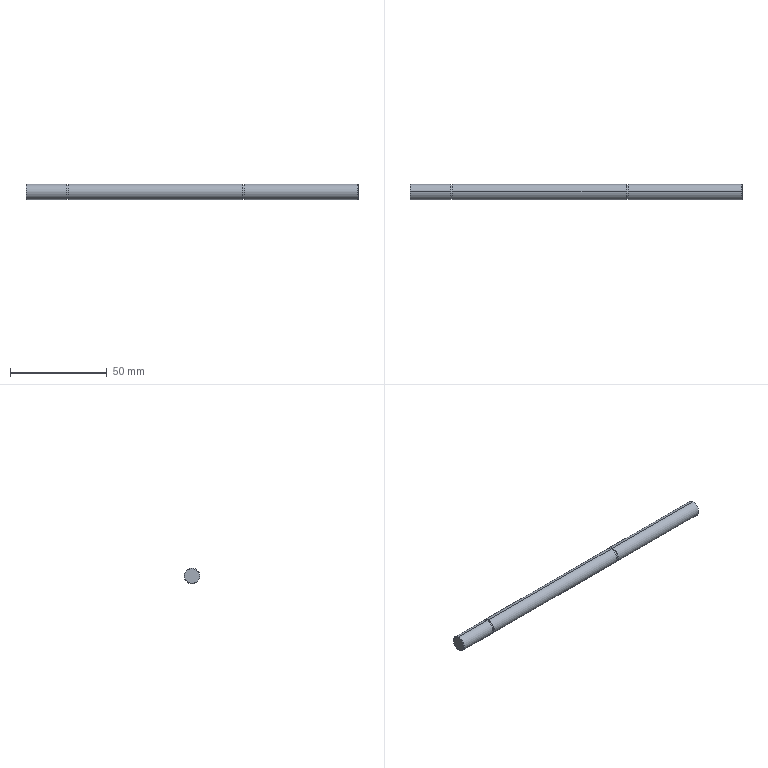Component | SolidWorks | 04-003DriveShaft-1 | 1 solid | 20 faces | box 172 x 8 x 8 mm | volume 8630 mm3 | cylinder 10 | plane 6 | cone 4 | commonest cylinder face diameters 8 x6 7.4 x4
build123d program:
from build123d import *

# Parameters (mm, degrees)
SKETCH1_R           = 4
BOSS_EXTRUDE1_DEPTH = 172
CHAMFER1_SIZE       = 0.2
SKETCH2_W           = 1
SKETCH2_H           = 0.3


with BuildPart() as part:
    # Sketch1 → Boss-Extrude1 (new body)
    with BuildSketch(Plane(origin=(0, 0, 0), x_dir=(0, 0, -1), z_dir=(1, 0, 0))):
        Circle(SKETCH1_R)
    extrude(amount=BOSS_EXTRUDE1_DEPTH)

    # Chamfer1
    chamfer1_edges = [part.edges().sort_by_distance(p)[0] for p in [
        (0, 0, 4),
        (172, 0, 4),
    ]]
    chamfer(chamfer1_edges, length=CHAMFER1_SIZE)

    # Sketch2 → Cut-Revolve1 (revolve, cut)
    with BuildSketch(Plane(origin=(0, 0, 0), x_dir=(1, 0, 0), z_dir=(0, 1, 0)), mode=Mode.PRIVATE) as cut_revolve1_sk:
        with Locations((21.5, 3.85)):
            Rectangle(SKETCH2_W, SKETCH2_H)
        with Locations((112.5, 3.85)):
            Rectangle(SKETCH2_W, SKETCH2_H)
    revolve(cut_revolve1_sk.sketch.rotate(Axis((0, 0, 0), (1, 0, 0)), 180), axis=Axis((0, 0, 0), (1, 0, 0)), mode=Mode.SUBTRACT)


solid = part.part

# Placed as in the assembly
solid = solid.moved(Location((-2.274, -5.336, 80.465), (0, 0, 0)))
STEP:
#1=COLOUR_RGB('',0.7922,0.8196,0.9333);
#2=FILL_AREA_STYLE_COLOUR('',#1);
#3=FILL_AREA_STYLE('',(#2));
#4=SURFACE_STYLE_FILL_AREA(#3);
#5=SURFACE_SIDE_STYLE('',(#4));
#6=SURFACE_STYLE_USAGE(.BOTH.,#5);
#7=PRESENTATION_STYLE_ASSIGNMENT((#6));
#8=CARTESIAN_POINT('',(6.674,-0.2215,3.011));
#9=VERTEX_POINT('',#8);
#10=CARTESIAN_POINT('',(6.674,-0.1986,3.325));
#11=VERTEX_POINT('',#10);
#12=CARTESIAN_POINT('',(6.674,-0.2101,3.168));
#13=DIRECTION('',(-1.,0.,0.));
#14=DIRECTION('',(0.,0.07282,0.9973));
#15=AXIS2_PLACEMENT_3D('',#12,#13,#14);
#16=CIRCLE('',#15,0.1575);
#17=EDGE_CURVE('',#9,#11,#16,.T.);
#18=ORIENTED_EDGE('',*,*,#17,.T.);
#19=CARTESIAN_POINT('',(4.359,-0.1986,3.325));
#20=VERTEX_POINT('',#19);
#21=CARTESIAN_POINT('',(6.682,-0.1986,3.325));
#22=DIRECTION('',(-1.,0.,0.));
#23=VECTOR('',#22,39.37);
#24=LINE('',#21,#23);
#25=EDGE_CURVE('',#11,#20,#24,.T.);
#26=ORIENTED_EDGE('',*,*,#25,.T.);
#27=CARTESIAN_POINT('',(4.359,-0.2215,3.011));
#28=VERTEX_POINT('',#27);
#29=CARTESIAN_POINT('',(4.359,-0.2101,3.168));
#30=DIRECTION('',(-1.,0.,0.));
#31=DIRECTION('',(0.,-0.07282,-0.9973));
#32=AXIS2_PLACEMENT_3D('',#29,#30,#31);
#33=CIRCLE('',#32,0.1575);
#34=EDGE_CURVE('',#28,#20,#33,.T.);
#35=ORIENTED_EDGE('',*,*,#34,.F.);
#36=CARTESIAN_POINT('',(6.682,-0.2215,3.011));
#37=DIRECTION('',(-1.,0.,0.));
#38=VECTOR('',#37,39.37);
#39=LINE('',#36,#38);
#40=EDGE_CURVE('',#9,#28,#39,.T.);
#41=ORIENTED_EDGE('',*,*,#40,.F.);
#42=EDGE_LOOP('',(#18,#26,#35,#41));
#43=FACE_OUTER_BOUND('',#42,.T.);
#44=CARTESIAN_POINT('',(6.682,-0.2101,3.168));
#45=DIRECTION('',(-1.,0.,0.));
#46=DIRECTION('',(0.,-0.07282,-0.9973));
#47=AXIS2_PLACEMENT_3D('',#44,#45,#46);
#48=CYLINDRICAL_SURFACE('',#47,0.1575);
#49=ADVANCED_FACE('',(#43),#48,.T.);
#50=CARTESIAN_POINT('',(6.682,-0.1992,3.317));
#51=VERTEX_POINT('',#50);
#52=CARTESIAN_POINT('',(6.682,-0.221,3.019));
#53=VERTEX_POINT('',#52);
#54=CARTESIAN_POINT('',(6.682,-0.2101,3.168));
#55=DIRECTION('',(1.,0.,0.));
#56=DIRECTION('',(0.,0.07282,0.9973));
#57=AXIS2_PLACEMENT_3D('',#54,#55,#56);
#58=CIRCLE('',#57,0.1496);
#59=EDGE_CURVE('',#51,#53,#58,.T.);
#60=ORIENTED_EDGE('',*,*,#59,.F.);
#61=CARTESIAN_POINT('',(6.682,-0.1992,3.317));
#62=DIRECTION('',(-0.7071,0.05149,0.7052));
#63=VECTOR('',#62,39.37);
#64=LINE('',#61,#63);
#65=EDGE_CURVE('',#51,#11,#64,.T.);
#66=ORIENTED_EDGE('',*,*,#65,.T.);
#67=ORIENTED_EDGE('',*,*,#17,.F.);
#68=CARTESIAN_POINT('',(6.682,-0.221,3.019));
#69=DIRECTION('',(-0.7071,-0.05149,-0.7052));
#70=VECTOR('',#69,39.37);
#71=LINE('',#68,#70);
#72=EDGE_CURVE('',#53,#9,#71,.T.);
#73=ORIENTED_EDGE('',*,*,#72,.F.);
#74=EDGE_LOOP('',(#60,#66,#67,#73));
#75=FACE_OUTER_BOUND('',#74,.T.);
#76=CARTESIAN_POINT('',(6.682,-0.2101,3.168));
#77=DIRECTION('',(-1.,0.,0.));
#78=DIRECTION('',(0.,-0.07282,-0.9973));
#79=AXIS2_PLACEMENT_3D('',#76,#77,#78);
#80=CONICAL_SURFACE('',#79,0.1496,0.7854);
#81=ADVANCED_FACE('',(#75),#80,.T.);
#82=CARTESIAN_POINT('',(4.359,-0.2207,3.023));
#83=VERTEX_POINT('',#82);
#84=CARTESIAN_POINT('',(4.359,-0.1995,3.313));
#85=VERTEX_POINT('',#84);
#86=CARTESIAN_POINT('',(4.359,-0.2101,3.168));
#87=DIRECTION('',(-1.,0.,0.));
#88=DIRECTION('',(0.,-0.07282,-0.9973));
#89=AXIS2_PLACEMENT_3D('',#86,#87,#88);
#90=CIRCLE('',#89,0.1457);
#91=EDGE_CURVE('',#83,#85,#90,.T.);
#92=ORIENTED_EDGE('',*,*,#91,.T.);
#93=CARTESIAN_POINT('',(4.32,-0.1995,3.313));
#94=VERTEX_POINT('',#93);
#95=CARTESIAN_POINT('',(-0.08951,-0.1995,3.313));
#96=DIRECTION('',(-1.,0.,0.));
#97=VECTOR('',#96,39.37);
#98=LINE('',#95,#97);
#99=EDGE_CURVE('',#85,#94,#98,.T.);
#100=ORIENTED_EDGE('',*,*,#99,.T.);
#101=CARTESIAN_POINT('',(4.32,-0.2207,3.023));
#102=VERTEX_POINT('',#101);
#103=CARTESIAN_POINT('',(4.32,-0.2101,3.168));
#104=DIRECTION('',(-1.,0.,0.));
#105=DIRECTION('',(0.,-0.07282,-0.9973));
#106=AXIS2_PLACEMENT_3D('',#103,#104,#105);
#107=CIRCLE('',#106,0.1457);
#108=EDGE_CURVE('',#102,#94,#107,.T.);
#109=ORIENTED_EDGE('',*,*,#108,.F.);
#110=CARTESIAN_POINT('',(-0.08951,-0.2207,3.023));
#111=DIRECTION('',(-1.,0.,0.));
#112=VECTOR('',#111,39.37);
#113=LINE('',#110,#112);
#114=EDGE_CURVE('',#83,#102,#113,.T.);
#115=ORIENTED_EDGE('',*,*,#114,.F.);
#116=EDGE_LOOP('',(#92,#100,#109,#115));
#117=FACE_OUTER_BOUND('',#116,.T.);
#118=CARTESIAN_POINT('',(-0.08951,-0.2101,3.168));
#119=DIRECTION('',(-1.,0.,0.));
#120=DIRECTION('',(0.,-0.07282,-0.9973));
#121=AXIS2_PLACEMENT_3D('',#118,#119,#120);
#122=CYLINDRICAL_SURFACE('',#121,0.1457);
#123=ADVANCED_FACE('',(#117),#122,.T.);
#124=CARTESIAN_POINT('',(4.32,-0.2215,3.011));
#125=VERTEX_POINT('',#124);
#126=CARTESIAN_POINT('',(4.32,-0.1986,3.325));
#127=VERTEX_POINT('',#126);
#128=CARTESIAN_POINT('',(4.32,-0.2101,3.168));
#129=DIRECTION('',(-1.,0.,0.));
#130=DIRECTION('',(0.,-0.07282,-0.9973));
#131=AXIS2_PLACEMENT_3D('',#128,#129,#130);
#132=CIRCLE('',#131,0.1575);
#133=EDGE_CURVE('',#125,#127,#132,.T.);
#134=ORIENTED_EDGE('',*,*,#133,.T.);
#135=CARTESIAN_POINT('',(0.7766,-0.1986,3.325));
#136=VERTEX_POINT('',#135);
#137=CARTESIAN_POINT('',(6.682,-0.1986,3.325));
#138=DIRECTION('',(-1.,0.,0.));
#139=VECTOR('',#138,39.37);
#140=LINE('',#137,#139);
#141=EDGE_CURVE('',#127,#136,#140,.T.);
#142=ORIENTED_EDGE('',*,*,#141,.T.);
#143=CARTESIAN_POINT('',(0.7766,-0.2215,3.011));
#144=VERTEX_POINT('',#143);
#145=CARTESIAN_POINT('',(0.7766,-0.2101,3.168));
#146=DIRECTION('',(-1.,0.,0.));
#147=DIRECTION('',(0.,-0.07282,-0.9973));
#148=AXIS2_PLACEMENT_3D('',#145,#146,#147);
#149=CIRCLE('',#148,0.1575);
#150=EDGE_CURVE('',#144,#136,#149,.T.);
#151=ORIENTED_EDGE('',*,*,#150,.F.);
#152=CARTESIAN_POINT('',(6.682,-0.2215,3.011));
#153=DIRECTION('',(-1.,0.,0.));
#154=VECTOR('',#153,39.37);
#155=LINE('',#152,#154);
#156=EDGE_CURVE('',#125,#144,#155,.T.);
#157=ORIENTED_EDGE('',*,*,#156,.F.);
#158=EDGE_LOOP('',(#134,#142,#151,#157));
#159=FACE_OUTER_BOUND('',#158,.T.);
#160=CARTESIAN_POINT('',(6.682,-0.2101,3.168));
#161=DIRECTION('',(-1.,0.,0.));
#162=DIRECTION('',(0.,-0.07282,-0.9973));
#163=AXIS2_PLACEMENT_3D('',#160,#161,#162);
#164=CYLINDRICAL_SURFACE('',#163,0.1575);
#165=ADVANCED_FACE('',(#159),#164,.T.);
#166=CARTESIAN_POINT('',(0.7766,-0.2207,3.023));
#167=VERTEX_POINT('',#166);
#168=CARTESIAN_POINT('',(0.7766,-0.1995,3.313));
#169=VERTEX_POINT('',#168);
#170=CARTESIAN_POINT('',(0.7766,-0.2101,3.168));
#171=DIRECTION('',(-1.,0.,0.));
#172=DIRECTION('',(0.,-0.07282,-0.9973));
#173=AXIS2_PLACEMENT_3D('',#170,#171,#172);
#174=CIRCLE('',#173,0.1457);
#175=EDGE_CURVE('',#167,#169,#174,.T.);
#176=ORIENTED_EDGE('',*,*,#175,.T.);
#177=CARTESIAN_POINT('',(0.7373,-0.1995,3.313));
#178=VERTEX_POINT('',#177);
#179=CARTESIAN_POINT('',(-0.08951,-0.1995,3.313));
#180=DIRECTION('',(-1.,0.,0.));
#181=VECTOR('',#180,39.37);
#182=LINE('',#179,#181);
#183=EDGE_CURVE('',#169,#178,#182,.T.);
#184=ORIENTED_EDGE('',*,*,#183,.T.);
#185=CARTESIAN_POINT('',(0.7373,-0.2207,3.023));
#186=VERTEX_POINT('',#185);
#187=CARTESIAN_POINT('',(0.7373,-0.2101,3.168));
#188=DIRECTION('',(-1.,0.,0.));
#189=DIRECTION('',(0.,-0.07282,-0.9973));
#190=AXIS2_PLACEMENT_3D('',#187,#188,#189);
#191=CIRCLE('',#190,0.1457);
#192=EDGE_CURVE('',#186,#178,#191,.T.);
#193=ORIENTED_EDGE('',*,*,#192,.F.);
#194=CARTESIAN_POINT('',(-0.08951,-0.2207,3.023));
#195=DIRECTION('',(-1.,0.,0.));
#196=VECTOR('',#195,39.37);
#197=LINE('',#194,#196);
#198=EDGE_CURVE('',#167,#186,#197,.T.);
#199=ORIENTED_EDGE('',*,*,#198,.F.);
#200=EDGE_LOOP('',(#176,#184,#193,#199));
#201=FACE_OUTER_BOUND('',#200,.T.);
#202=CARTESIAN_POINT('',(-0.08951,-0.2101,3.168));
#203=DIRECTION('',(-1.,0.,0.));
#204=DIRECTION('',(0.,-0.07282,-0.9973));
#205=AXIS2_PLACEMENT_3D('',#202,#203,#204);
#206=CYLINDRICAL_SURFACE('',#205,0.1457);
#207=ADVANCED_FACE('',(#201),#206,.T.);
#208=CARTESIAN_POINT('',(-0.08951,-0.221,3.019));
#209=VERTEX_POINT('',#208);
#210=CARTESIAN_POINT('',(-0.08951,-0.1992,3.317));
#211=VERTEX_POINT('',#210);
#212=CARTESIAN_POINT('',(-0.08951,-0.2101,3.168));
#213=DIRECTION('',(-1.,0.,0.));
#214=DIRECTION('',(0.,0.07282,0.9973));
#215=AXIS2_PLACEMENT_3D('',#212,#213,#214);
#216=CIRCLE('',#215,0.1496);
#217=EDGE_CURVE('',#209,#211,#216,.T.);
#218=ORIENTED_EDGE('',*,*,#217,.F.);
#219=CARTESIAN_POINT('',(-0.08164,-0.2215,3.011));
#220=VERTEX_POINT('',#219);
#221=CARTESIAN_POINT('',(-0.08164,-0.2215,3.011));
#222=DIRECTION('',(0.7071,-0.05149,-0.7052));
#223=VECTOR('',#222,39.37);
#224=LINE('',#221,#223);
#225=EDGE_CURVE('',#209,#220,#224,.T.);
#226=ORIENTED_EDGE('',*,*,#225,.T.);
#227=CARTESIAN_POINT('',(-0.08164,-0.1986,3.325));
#228=VERTEX_POINT('',#227);
#229=CARTESIAN_POINT('',(-0.08164,-0.2101,3.168));
#230=DIRECTION('',(1.,0.,0.));
#231=DIRECTION('',(0.,0.07282,0.9973));
#232=AXIS2_PLACEMENT_3D('',#229,#230,#231);
#233=CIRCLE('',#232,0.1575);
#234=EDGE_CURVE('',#228,#220,#233,.T.);
#235=ORIENTED_EDGE('',*,*,#234,.F.);
#236=CARTESIAN_POINT('',(-0.08164,-0.1986,3.325));
#237=DIRECTION('',(0.7071,0.05149,0.7052));
#238=VECTOR('',#237,39.37);
#239=LINE('',#236,#238);
#240=EDGE_CURVE('',#211,#228,#239,.T.);
#241=ORIENTED_EDGE('',*,*,#240,.F.);
#242=EDGE_LOOP('',(#218,#226,#235,#241));
#243=FACE_OUTER_BOUND('',#242,.T.);
#244=CARTESIAN_POINT('',(-0.08164,-0.2101,3.168));
#245=DIRECTION('',(1.,0.,0.));
#246=DIRECTION('',(0.,0.07282,0.9973));
#247=AXIS2_PLACEMENT_3D('',#244,#245,#246);
#248=CONICAL_SURFACE('',#247,0.1575,0.7854);
#249=ADVANCED_FACE('',(#243),#248,.T.);
#250=CARTESIAN_POINT('',(0.7373,-0.2215,3.011));
#251=VERTEX_POINT('',#250);
#252=CARTESIAN_POINT('',(0.7373,-0.1986,3.325));
#253=VERTEX_POINT('',#252);
#254=CARTESIAN_POINT('',(0.7373,-0.2101,3.168));
#255=DIRECTION('',(-1.,0.,0.));
#256=DIRECTION('',(0.,-0.07282,-0.9973));
#257=AXIS2_PLACEMENT_3D('',#254,#255,#256);
#258=CIRCLE('',#257,0.1575);
#259=EDGE_CURVE('',#251,#253,#258,.T.);
#260=ORIENTED_EDGE('',*,*,#259,.T.);
#261=CARTESIAN_POINT('',(6.682,-0.1986,3.325));
#262=DIRECTION('',(-1.,0.,0.));
#263=VECTOR('',#262,39.37);
#264=LINE('',#261,#263);
#265=EDGE_CURVE('',#253,#228,#264,.T.);
#266=ORIENTED_EDGE('',*,*,#265,.T.);
#267=ORIENTED_EDGE('',*,*,#234,.T.);
#268=CARTESIAN_POINT('',(6.682,-0.2215,3.011));
#269=DIRECTION('',(-1.,0.,0.));
#270=VECTOR('',#269,39.37);
#271=LINE('',#268,#270);
#272=EDGE_CURVE('',#251,#220,#271,.T.);
#273=ORIENTED_EDGE('',*,*,#272,.F.);
#274=EDGE_LOOP('',(#260,#266,#267,#273));
#275=FACE_OUTER_BOUND('',#274,.T.);
#276=CARTESIAN_POINT('',(6.682,-0.2101,3.168));
#277=DIRECTION('',(-1.,0.,0.));
#278=DIRECTION('',(0.,-0.07282,-0.9973));
#279=AXIS2_PLACEMENT_3D('',#276,#277,#278);
#280=CYLINDRICAL_SURFACE('',#279,0.1575);
#281=ADVANCED_FACE('',(#275),#280,.T.);
#282=ORIENTED_EDGE('',*,*,#265,.F.);
#283=CARTESIAN_POINT('',(0.7373,-0.2101,3.168));
#284=DIRECTION('',(-1.,0.,0.));
#285=DIRECTION('',(0.,-0.07282,-0.9973));
#286=AXIS2_PLACEMENT_3D('',#283,#284,#285);
#287=CIRCLE('',#286,0.1575);
#288=EDGE_CURVE('',#253,#251,#287,.T.);
#289=ORIENTED_EDGE('',*,*,#288,.T.);
#290=ORIENTED_EDGE('',*,*,#272,.T.);
#291=CARTESIAN_POINT('',(-0.08164,-0.2101,3.168));
#292=DIRECTION('',(1.,0.,0.));
#293=DIRECTION('',(0.,0.07282,0.9973));
#294=AXIS2_PLACEMENT_3D('',#291,#292,#293);
#295=CIRCLE('',#294,0.1575);
#296=EDGE_CURVE('',#220,#228,#295,.T.);
#297=ORIENTED_EDGE('',*,*,#296,.T.);
#298=EDGE_LOOP('',(#282,#289,#290,#297));
#299=FACE_OUTER_BOUND('',#298,.T.);
#300=CARTESIAN_POINT('',(6.682,-0.2101,3.168));
#301=DIRECTION('',(-1.,0.,0.));
#302=DIRECTION('',(0.,-0.07282,-0.9973));
#303=AXIS2_PLACEMENT_3D('',#300,#301,#302);
#304=CYLINDRICAL_SURFACE('',#303,0.1575);
#305=ADVANCED_FACE('',(#299),#304,.T.);
#306=CARTESIAN_POINT('',(-0.08951,-0.2101,3.168));
#307=DIRECTION('',(-1.,0.,0.));
#308=DIRECTION('',(0.,0.07282,0.9973));
#309=AXIS2_PLACEMENT_3D('',#306,#307,#308);
#310=CIRCLE('',#309,0.1496);
#311=EDGE_CURVE('',#211,#209,#310,.T.);
#312=ORIENTED_EDGE('',*,*,#311,.T.);
#313=ORIENTED_EDGE('',*,*,#217,.T.);
#314=EDGE_LOOP('',(#312,#313));
#315=FACE_OUTER_BOUND('',#314,.T.);
#316=CARTESIAN_POINT('',(-0.08951,-0.2101,3.168));
#317=DIRECTION('',(1.,0.,0.));
#318=DIRECTION('',(0.,0.07282,0.9973));
#319=AXIS2_PLACEMENT_3D('',#316,#317,#318);
#320=PLANE('',#319);
#321=ADVANCED_FACE('',(#315),#320,.F.);
#322=ORIENTED_EDGE('',*,*,#225,.F.);
#323=ORIENTED_EDGE('',*,*,#311,.F.);
#324=ORIENTED_EDGE('',*,*,#240,.T.);
#325=ORIENTED_EDGE('',*,*,#296,.F.);
#326=EDGE_LOOP('',(#322,#323,#324,#325));
#327=FACE_OUTER_BOUND('',#326,.T.);
#328=CARTESIAN_POINT('',(-0.08164,-0.2101,3.168));
#329=DIRECTION('',(1.,0.,0.));
#330=DIRECTION('',(0.,0.07282,0.9973));
#331=AXIS2_PLACEMENT_3D('',#328,#329,#330);
#332=CONICAL_SURFACE('',#331,0.1575,0.7854);
#333=ADVANCED_FACE('',(#327),#332,.T.);
#334=ORIENTED_EDGE('',*,*,#192,.T.);
#335=CARTESIAN_POINT('',(0.7373,-0.2101,3.168));
#336=DIRECTION('',(-1.,0.,0.));
#337=DIRECTION('',(0.,-0.07282,-0.9973));
#338=AXIS2_PLACEMENT_3D('',#335,#336,#337);
#339=CIRCLE('',#338,0.1457);
#340=EDGE_CURVE('',#178,#186,#339,.T.);
#341=ORIENTED_EDGE('',*,*,#340,.T.);
#342=EDGE_LOOP('',(#334,#341));
#343=FACE_BOUND('',#342,.T.);
#344=ORIENTED_EDGE('',*,*,#259,.F.);
#345=ORIENTED_EDGE('',*,*,#288,.F.);
#346=EDGE_LOOP('',(#344,#345));
#347=FACE_OUTER_BOUND('',#346,.T.);
#348=CARTESIAN_POINT('',(0.7373,-0.1986,3.325));
#349=DIRECTION('',(1.,0.,0.));
#350=DIRECTION('',(0.,0.07282,0.9973));
#351=AXIS2_PLACEMENT_3D('',#348,#349,#350);
#352=PLANE('',#351);
#353=ADVANCED_FACE('',(#343,#347),#352,.T.);
#354=ORIENTED_EDGE('',*,*,#183,.F.);
#355=CARTESIAN_POINT('',(0.7766,-0.2101,3.168));
#356=DIRECTION('',(-1.,0.,0.));
#357=DIRECTION('',(0.,-0.07282,-0.9973));
#358=AXIS2_PLACEMENT_3D('',#355,#356,#357);
#359=CIRCLE('',#358,0.1457);
#360=EDGE_CURVE('',#169,#167,#359,.T.);
#361=ORIENTED_EDGE('',*,*,#360,.T.);
#362=ORIENTED_EDGE('',*,*,#198,.T.);
#363=ORIENTED_EDGE('',*,*,#340,.F.);
#364=EDGE_LOOP('',(#354,#361,#362,#363));
#365=FACE_OUTER_BOUND('',#364,.T.);
#366=CARTESIAN_POINT('',(-0.08951,-0.2101,3.168));
#367=DIRECTION('',(-1.,0.,0.));
#368=DIRECTION('',(0.,-0.07282,-0.9973));
#369=AXIS2_PLACEMENT_3D('',#366,#367,#368);
#370=CYLINDRICAL_SURFACE('',#369,0.1457);
#371=ADVANCED_FACE('',(#365),#370,.T.);
#372=ORIENTED_EDGE('',*,*,#150,.T.);
#373=CARTESIAN_POINT('',(0.7766,-0.2101,3.168));
#374=DIRECTION('',(-1.,0.,0.));
#375=DIRECTION('',(0.,-0.07282,-0.9973));
#376=AXIS2_PLACEMENT_3D('',#373,#374,#375);
#377=CIRCLE('',#376,0.1575);
#378=EDGE_CURVE('',#136,#144,#377,.T.);
#379=ORIENTED_EDGE('',*,*,#378,.T.);
#380=EDGE_LOOP('',(#372,#379));
#381=FACE_OUTER_BOUND('',#380,.T.);
#382=ORIENTED_EDGE('',*,*,#175,.F.);
#383=ORIENTED_EDGE('',*,*,#360,.F.);
#384=EDGE_LOOP('',(#382,#383));
#385=FACE_BOUND('',#384,.T.);
#386=CARTESIAN_POINT('',(0.7766,-0.1986,3.325));
#387=DIRECTION('',(-1.,0.,0.));
#388=DIRECTION('',(0.,-0.07282,-0.9973));
#389=AXIS2_PLACEMENT_3D('',#386,#387,#388);
#390=PLANE('',#389);
#391=ADVANCED_FACE('',(#381,#385),#390,.T.);
#392=ORIENTED_EDGE('',*,*,#141,.F.);
#393=CARTESIAN_POINT('',(4.32,-0.2101,3.168));
#394=DIRECTION('',(-1.,0.,0.));
#395=DIRECTION('',(0.,-0.07282,-0.9973));
#396=AXIS2_PLACEMENT_3D('',#393,#394,#395);
#397=CIRCLE('',#396,0.1575);
#398=EDGE_CURVE('',#127,#125,#397,.T.);
#399=ORIENTED_EDGE('',*,*,#398,.T.);
#400=ORIENTED_EDGE('',*,*,#156,.T.);
#401=ORIENTED_EDGE('',*,*,#378,.F.);
#402=EDGE_LOOP('',(#392,#399,#400,#401));
#403=FACE_OUTER_BOUND('',#402,.T.);
#404=CARTESIAN_POINT('',(6.682,-0.2101,3.168));
#405=DIRECTION('',(-1.,0.,0.));
#406=DIRECTION('',(0.,-0.07282,-0.9973));
#407=AXIS2_PLACEMENT_3D('',#404,#405,#406);
#408=CYLINDRICAL_SURFACE('',#407,0.1575);
#409=ADVANCED_FACE('',(#403),#408,.T.);
#410=ORIENTED_EDGE('',*,*,#108,.T.);
#411=CARTESIAN_POINT('',(4.32,-0.2101,3.168));
#412=DIRECTION('',(-1.,0.,0.));
#413=DIRECTION('',(0.,-0.07282,-0.9973));
#414=AXIS2_PLACEMENT_3D('',#411,#412,#413);
#415=CIRCLE('',#414,0.1457);
#416=EDGE_CURVE('',#94,#102,#415,.T.);
#417=ORIENTED_EDGE('',*,*,#416,.T.);
#418=EDGE_LOOP('',(#410,#417));
#419=FACE_BOUND('',#418,.T.);
#420=ORIENTED_EDGE('',*,*,#133,.F.);
#421=ORIENTED_EDGE('',*,*,#398,.F.);
#422=EDGE_LOOP('',(#420,#421));
#423=FACE_OUTER_BOUND('',#422,.T.);
#424=CARTESIAN_POINT('',(4.32,-0.1986,3.325));
#425=DIRECTION('',(1.,0.,0.));
#426=DIRECTION('',(0.,0.07282,0.9973));
#427=AXIS2_PLACEMENT_3D('',#424,#425,#426);
#428=PLANE('',#427);
#429=ADVANCED_FACE('',(#419,#423),#428,.T.);
#430=ORIENTED_EDGE('',*,*,#99,.F.);
#431=CARTESIAN_POINT('',(4.359,-0.2101,3.168));
#432=DIRECTION('',(-1.,0.,0.));
#433=DIRECTION('',(0.,-0.07282,-0.9973));
#434=AXIS2_PLACEMENT_3D('',#431,#432,#433);
#435=CIRCLE('',#434,0.1457);
#436=EDGE_CURVE('',#85,#83,#435,.T.);
#437=ORIENTED_EDGE('',*,*,#436,.T.);
#438=ORIENTED_EDGE('',*,*,#114,.T.);
#439=ORIENTED_EDGE('',*,*,#416,.F.);
#440=EDGE_LOOP('',(#430,#437,#438,#439));
#441=FACE_OUTER_BOUND('',#440,.T.);
#442=CARTESIAN_POINT('',(-0.08951,-0.2101,3.168));
#443=DIRECTION('',(-1.,0.,0.));
#444=DIRECTION('',(0.,-0.07282,-0.9973));
#445=AXIS2_PLACEMENT_3D('',#442,#443,#444);
#446=CYLINDRICAL_SURFACE('',#445,0.1457);
#447=ADVANCED_FACE('',(#441),#446,.T.);
#448=ORIENTED_EDGE('',*,*,#34,.T.);
#449=CARTESIAN_POINT('',(4.359,-0.2101,3.168));
#450=DIRECTION('',(-1.,0.,0.));
#451=DIRECTION('',(0.,-0.07282,-0.9973));
#452=AXIS2_PLACEMENT_3D('',#449,#450,#451);
#453=CIRCLE('',#452,0.1575);
#454=EDGE_CURVE('',#20,#28,#453,.T.);
#455=ORIENTED_EDGE('',*,*,#454,.T.);
#456=EDGE_LOOP('',(#448,#455));
#457=FACE_OUTER_BOUND('',#456,.T.);
#458=ORIENTED_EDGE('',*,*,#91,.F.);
#459=ORIENTED_EDGE('',*,*,#436,.F.);
#460=EDGE_LOOP('',(#458,#459));
#461=FACE_BOUND('',#460,.T.);
#462=CARTESIAN_POINT('',(4.359,-0.1986,3.325));
#463=DIRECTION('',(-1.,0.,0.));
#464=DIRECTION('',(0.,-0.07282,-0.9973));
#465=AXIS2_PLACEMENT_3D('',#462,#463,#464);
#466=PLANE('',#465);
#467=ADVANCED_FACE('',(#457,#461),#466,.T.);
#468=CARTESIAN_POINT('',(6.682,-0.2101,3.168));
#469=DIRECTION('',(1.,0.,0.));
#470=DIRECTION('',(0.,0.07282,0.9973));
#471=AXIS2_PLACEMENT_3D('',#468,#469,#470);
#472=CIRCLE('',#471,0.1496);
#473=EDGE_CURVE('',#53,#51,#472,.T.);
#474=ORIENTED_EDGE('',*,*,#473,.T.);
#475=ORIENTED_EDGE('',*,*,#59,.T.);
#476=EDGE_LOOP('',(#474,#475));
#477=FACE_OUTER_BOUND('',#476,.T.);
#478=CARTESIAN_POINT('',(6.682,-0.2101,3.168));
#479=DIRECTION('',(1.,0.,0.));
#480=DIRECTION('',(0.,0.07282,0.9973));
#481=AXIS2_PLACEMENT_3D('',#478,#479,#480);
#482=PLANE('',#481);
#483=ADVANCED_FACE('',(#477),#482,.T.);
#484=ORIENTED_EDGE('',*,*,#65,.F.);
#485=ORIENTED_EDGE('',*,*,#473,.F.);
#486=ORIENTED_EDGE('',*,*,#72,.T.);
#487=CARTESIAN_POINT('',(6.674,-0.2101,3.168));
#488=DIRECTION('',(-1.,0.,0.));
#489=DIRECTION('',(0.,0.07282,0.9973));
#490=AXIS2_PLACEMENT_3D('',#487,#488,#489);
#491=CIRCLE('',#490,0.1575);
#492=EDGE_CURVE('',#11,#9,#491,.T.);
#493=ORIENTED_EDGE('',*,*,#492,.F.);
#494=EDGE_LOOP('',(#484,#485,#486,#493));
#495=FACE_OUTER_BOUND('',#494,.T.);
#496=CARTESIAN_POINT('',(6.682,-0.2101,3.168));
#497=DIRECTION('',(-1.,0.,0.));
#498=DIRECTION('',(0.,-0.07282,-0.9973));
#499=AXIS2_PLACEMENT_3D('',#496,#497,#498);
#500=CONICAL_SURFACE('',#499,0.1496,0.7854);
#501=ADVANCED_FACE('',(#495),#500,.T.);
#502=ORIENTED_EDGE('',*,*,#25,.F.);
#503=ORIENTED_EDGE('',*,*,#492,.T.);
#504=ORIENTED_EDGE('',*,*,#40,.T.);
#505=ORIENTED_EDGE('',*,*,#454,.F.);
#506=EDGE_LOOP('',(#502,#503,#504,#505));
#507=FACE_OUTER_BOUND('',#506,.T.);
#508=CARTESIAN_POINT('',(6.682,-0.2101,3.168));
#509=DIRECTION('',(-1.,0.,0.));
#510=DIRECTION('',(0.,-0.07282,-0.9973));
#511=AXIS2_PLACEMENT_3D('',#508,#509,#510);
#512=CYLINDRICAL_SURFACE('',#511,0.1575);
#513=ADVANCED_FACE('',(#507),#512,.T.);
#514=CLOSED_SHELL('',(#49,#81,#123,#165,#207,#249,#281,#305,#321,#333,#353,#371,#391,#409,#429,#447,#467,#483,#501,#513));
#515=MANIFOLD_SOLID_BREP('',#514);
#516=STYLED_ITEM('',(#7),#515);
#517=(LENGTH_UNIT()NAMED_UNIT(*)SI_UNIT($,.METRE.));
#518=LENGTH_MEASURE_WITH_UNIT(LENGTH_MEASURE(0.0254),#517);
#519=DIMENSIONAL_EXPONENTS(1.,0.,0.,0.,0.,0.,0.);
#520=(CONVERSION_BASED_UNIT('',#518)LENGTH_UNIT()NAMED_UNIT(#519));
#521=UNCERTAINTY_MEASURE_WITH_UNIT(LENGTH_MEASURE(0.00001),#520,'','');
#522=(NAMED_UNIT(*)PLANE_ANGLE_UNIT()SI_UNIT($,.RADIAN.));
#523=(NAMED_UNIT(*)SI_UNIT($,.STERADIAN.)SOLID_ANGLE_UNIT());
#524=(GEOMETRIC_REPRESENTATION_CONTEXT(3)GLOBAL_UNCERTAINTY_ASSIGNED_CONTEXT((#521))GLOBAL_UNIT_ASSIGNED_CONTEXT((#520,#522,#523))REPRESENTATION_CONTEXT('',''));
#525=MECHANICAL_DESIGN_GEOMETRIC_PRESENTATION_REPRESENTATION('',(#516),#524);
#526=CARTESIAN_POINT('',(0.,0.,0.));
#527=DIRECTION('',(0.,0.,1.));
#528=DIRECTION('',(1.,0.,0.));
#529=AXIS2_PLACEMENT_3D('',#526,#527,#528);
#530=(LENGTH_UNIT()NAMED_UNIT(*)SI_UNIT($,.METRE.));
#531=LENGTH_MEASURE_WITH_UNIT(LENGTH_MEASURE(0.0254),#530);
#532=DIMENSIONAL_EXPONENTS(1.,0.,0.,0.,0.,0.,0.);
#533=(CONVERSION_BASED_UNIT('',#531)LENGTH_UNIT()NAMED_UNIT(#532));
#534=UNCERTAINTY_MEASURE_WITH_UNIT(LENGTH_MEASURE(0.00001),#533,'','');
#535=(NAMED_UNIT(*)PLANE_ANGLE_UNIT()SI_UNIT($,.RADIAN.));
#536=(NAMED_UNIT(*)SI_UNIT($,.STERADIAN.)SOLID_ANGLE_UNIT());
#537=(GEOMETRIC_REPRESENTATION_CONTEXT(3)GLOBAL_UNCERTAINTY_ASSIGNED_CONTEXT((#534))GLOBAL_UNIT_ASSIGNED_CONTEXT((#533,#535,#536))REPRESENTATION_CONTEXT('',''));
#538=ADVANCED_BREP_SHAPE_REPRESENTATION('',(#515,#529),#537);
#539=PRESENTATION_LAYER_ASSIGNMENT('','',(#516));